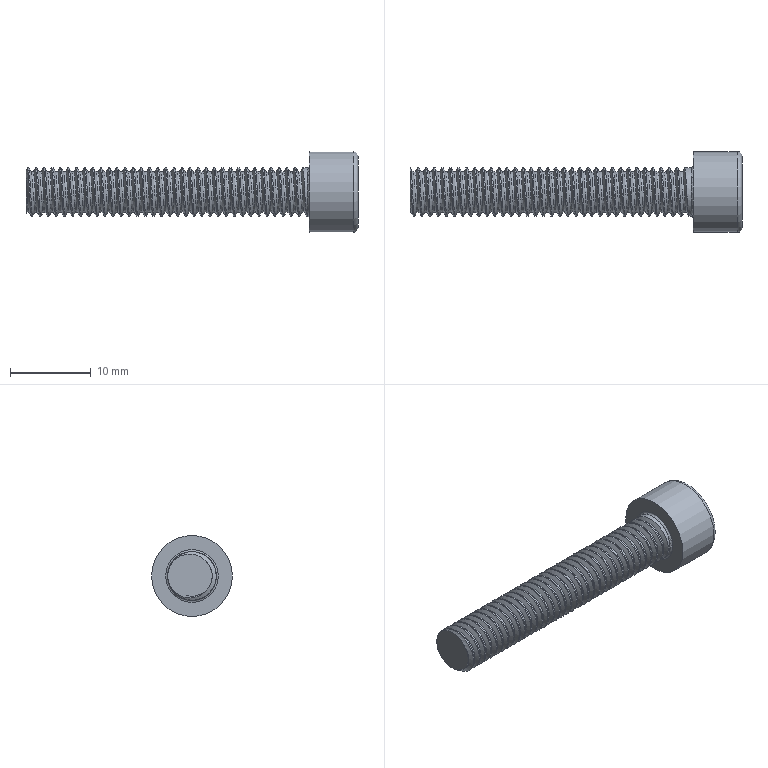Component | NX | M6X12_HEX_BOLT_12 | 1 solid | 30 faces | volume 1183 mm3 | plane 16 | cone 7 | cylinder 3 | torus 2 | spline 2 | commonest cylinder face diameters 6 x1 10 x1 5 x1